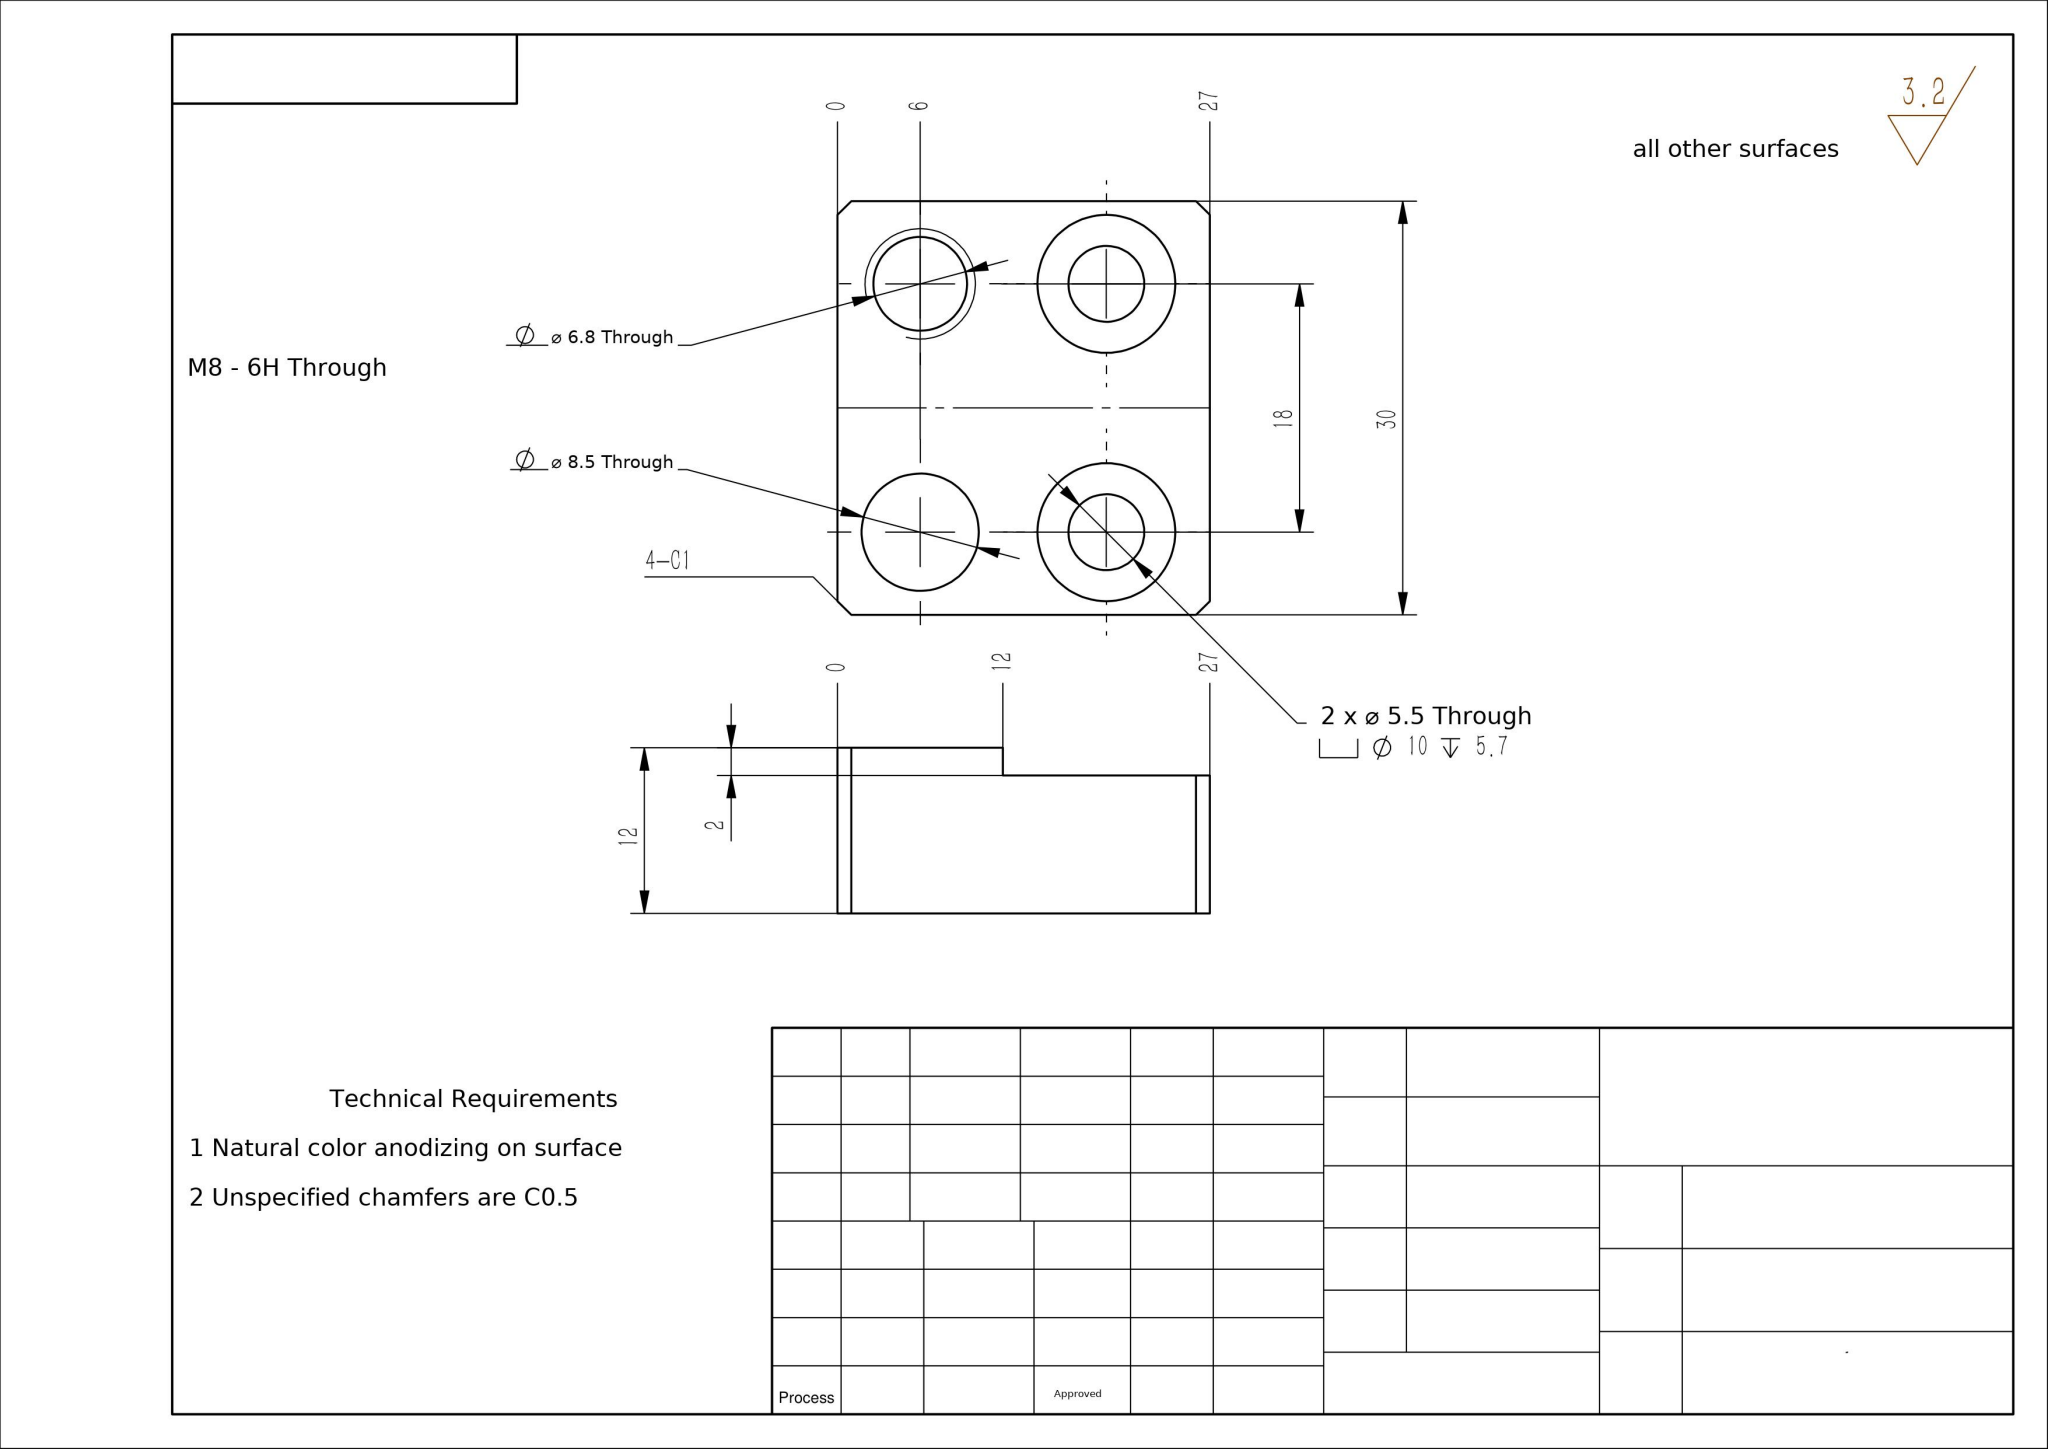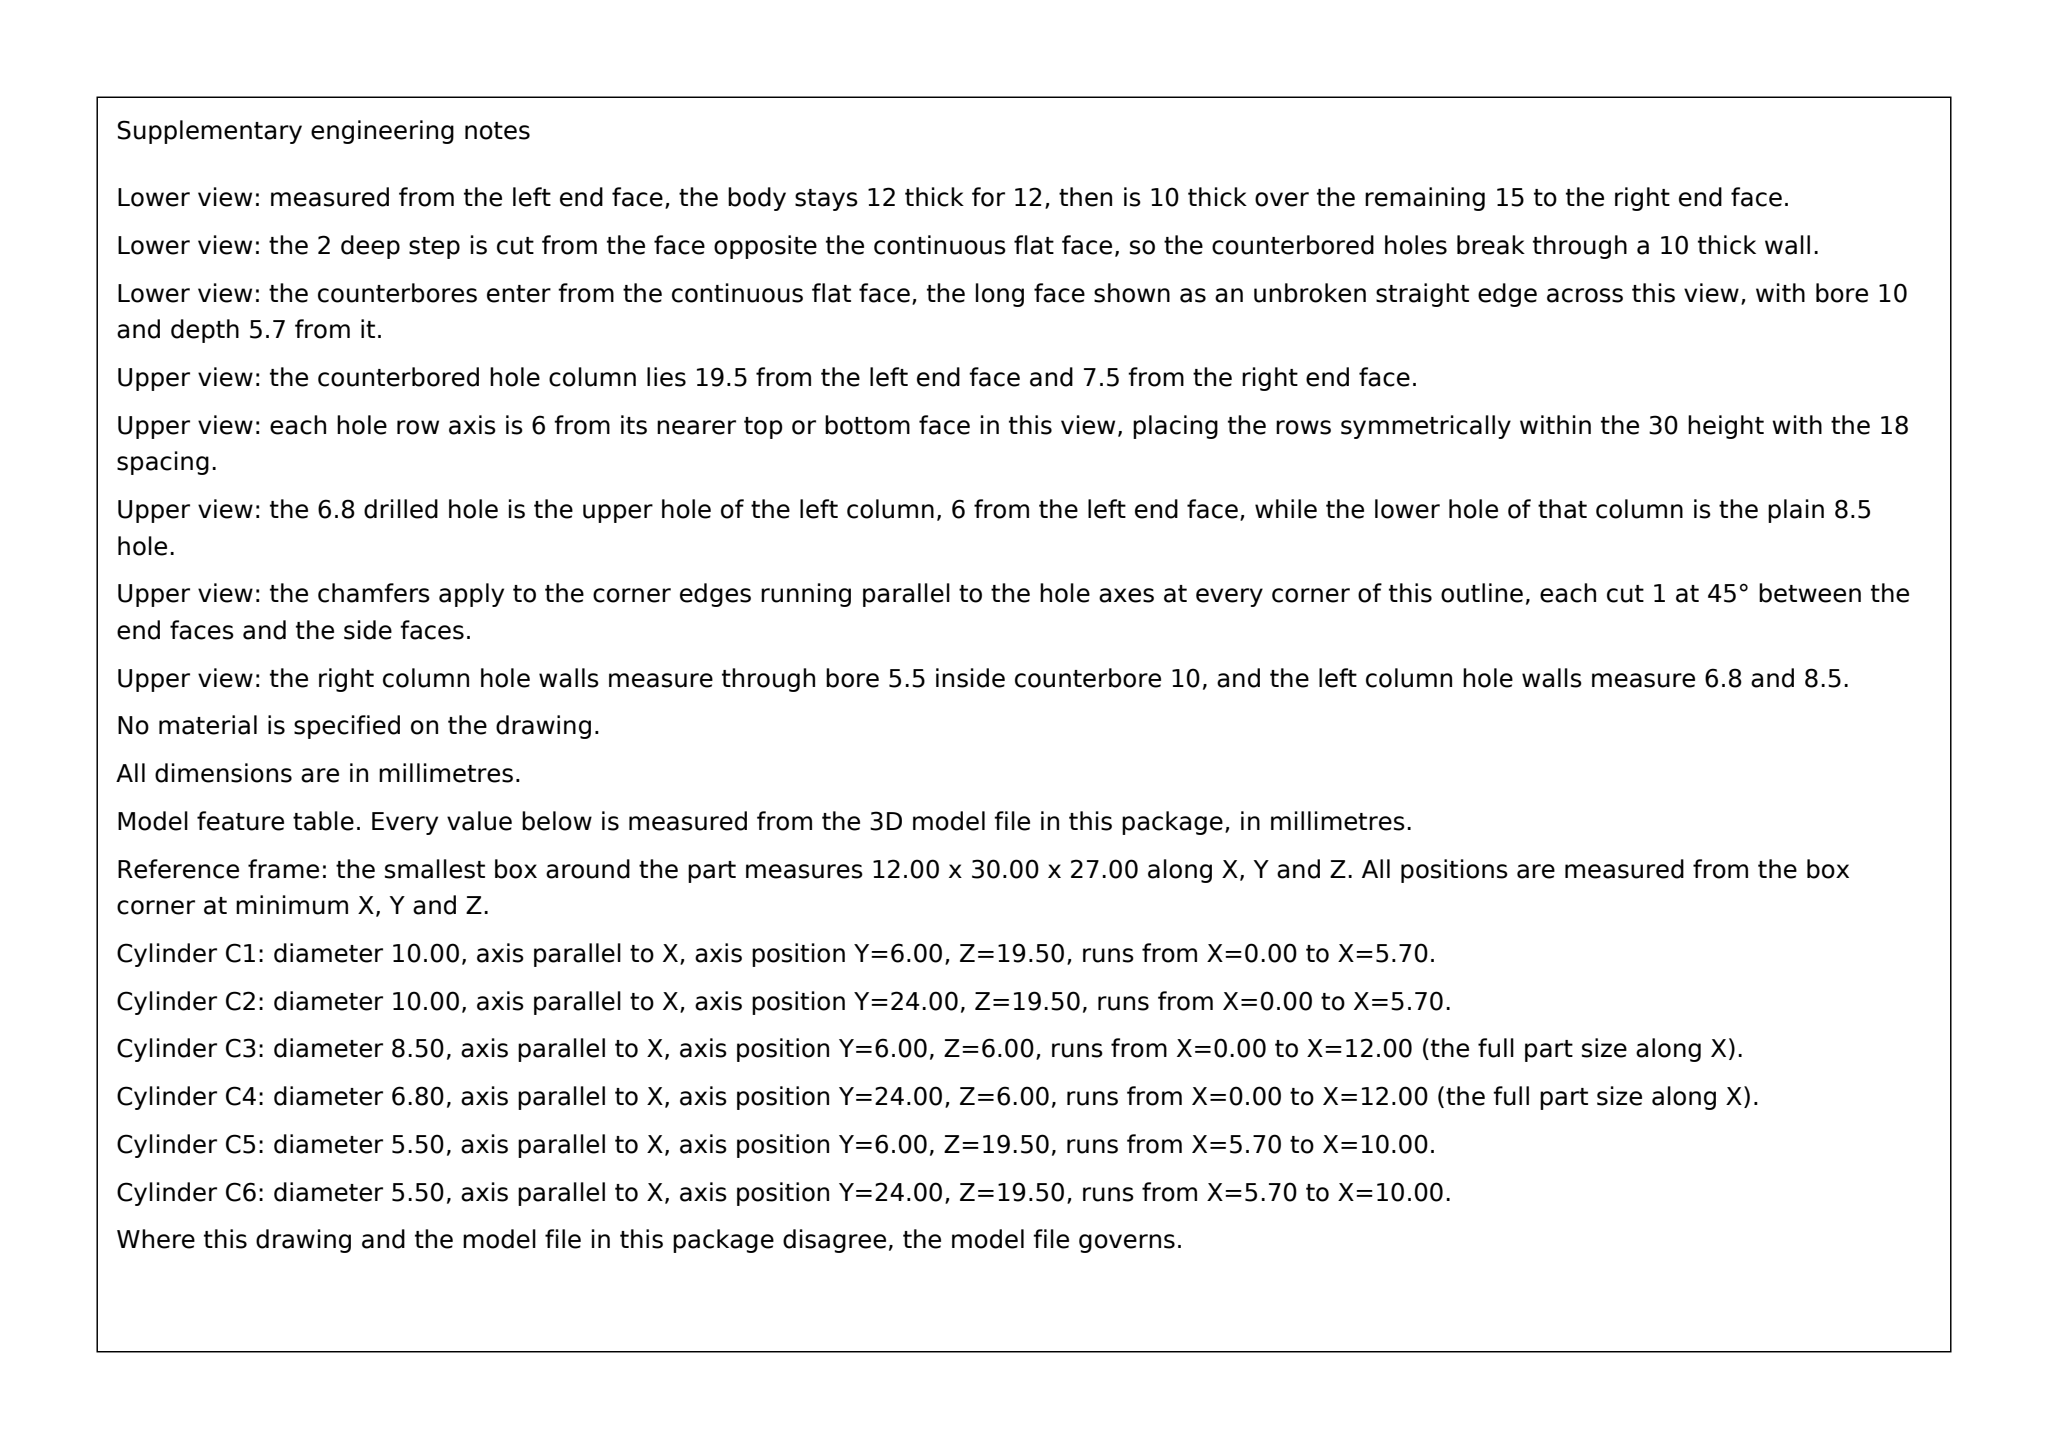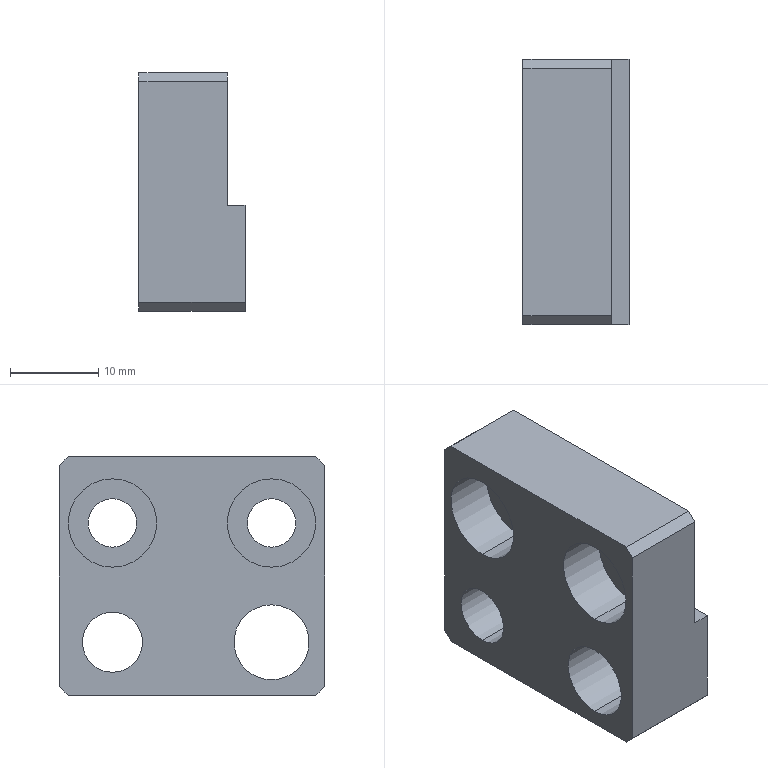Part | SolidWorks | mm | 1 solid | 26 faces | box 12 x 30 x 27 mm | volume 6582 mm3 | plane 14 | cylinder 12 | commonest cylinder face diameters 10 x4 5.5 x4 8.5 x2 6.8 x2
Drawing notes:
2 X Ø5.5/Ø10 C'BORE CL AT ORD 19.5 FROM 0 DATUM EDGE | from the solid: Ø10 & Ø5.5 bores, x-axis, axis_pos z=19.5 (y=6.0 & 24.0); bbox z 0-27
build123d program:
from build123d import *

# Parameters (mm, degrees)
BOSS_EXTRUDE1_DEPTH                               = 30
HOLE_SIZE_ACCORDING_TO_HEXAGON_SOCKET_D           = 5.5
HOLE_SIZE_ACCORDING_TO_HEXAGON_SOCKET_CBORE_D     = 10
HOLE_SIZE_ACCORDING_TO_HEXAGON_SOCKET_CBORE_DEPTH = 5.7
M8_TAPPED_HOLE1_D                                 = 6.8
F_8_5_8_5_DIAMETER_HOLE1_D                        = 8.5
CHAMFER1_SIZE                                     = 1


with BuildPart() as part:
    # Sketch1 → Boss-Extrude1 (new body)
    with BuildSketch(Plane(origin=(0, 0, 0), x_dir=(1, 0, 0), z_dir=(0, 1, 0))):
        Polygon((-23.167, 25.917), (-11.167, 25.917), (-11.167, 13.917), (-13.167, 13.917), (-13.167, -1.083), (-23.167, -1.083), align=None)
    extrude(amount=BOSS_EXTRUDE1_DEPTH)

    # Hole Size _ according to_ Hexagon Socket (through all)
    with Locations(Plane.ZY.offset(23.167)):
        with Locations((-6.417, 6), (-6.417, 24)):
            CounterBoreHole(HOLE_SIZE_ACCORDING_TO_HEXAGON_SOCKET_D / 2, HOLE_SIZE_ACCORDING_TO_HEXAGON_SOCKET_CBORE_D / 2, HOLE_SIZE_ACCORDING_TO_HEXAGON_SOCKET_CBORE_DEPTH)

    # M8 Tapped Hole1 (through all)
    with Locations(Plane.ZY.offset(23.167)):
        with Locations((-19.917, 24)):
            Hole(M8_TAPPED_HOLE1_D / 2)

    # 8.5 _8.5_ Diameter Hole1 (through all)
    with Locations(Plane.ZY.offset(23.167)):
        with Locations((-19.917, 6)):
            Hole(F_8_5_8_5_DIAMETER_HOLE1_D / 2)

    # Chamfer1
    chamfer1_edges = [part.edges().sort_by_distance(p)[0] for p in [
        (-17.167, 30, -25.917),
        (-17.167, 0, -25.917),
        (-18.167, 30, 1.083),
        (-18.167, 0, 1.083),
    ]]
    chamfer(chamfer1_edges, length=CHAMFER1_SIZE)


solid = part.part
STEP:
#1=CARTESIAN_POINT('',(-11.167,6.,-24.167));
#2=VERTEX_POINT('',#1);
#3=CARTESIAN_POINT('',(-11.167,6.,-15.667));
#4=VERTEX_POINT('',#3);
#5=CARTESIAN_POINT('',(-11.167,6.,-19.917));
#6=DIRECTION('',(-1.,0.,0.));
#7=DIRECTION('',(0.,0.,1.));
#8=AXIS2_PLACEMENT_3D('',#5,#6,#7);
#9=CIRCLE('',#8,4.25);
#10=EDGE_CURVE('',#2,#4,#9,.T.);
#11=ORIENTED_EDGE('',*,*,#10,.F.);
#12=CARTESIAN_POINT('',(-23.167,6.,-24.167));
#13=VERTEX_POINT('',#12);
#14=CARTESIAN_POINT('',(-23.167,6.,-24.167));
#15=DIRECTION('',(-1.,0.,0.));
#16=VECTOR('',#15,1000.);
#17=LINE('',#14,#16);
#18=EDGE_CURVE('',#2,#13,#17,.T.);
#19=ORIENTED_EDGE('',*,*,#18,.T.);
#20=CARTESIAN_POINT('',(-23.167,6.,-15.667));
#21=VERTEX_POINT('',#20);
#22=CARTESIAN_POINT('',(-23.167,6.,-19.917));
#23=DIRECTION('',(-1.,0.,0.));
#24=DIRECTION('',(0.,0.,1.));
#25=AXIS2_PLACEMENT_3D('',#22,#23,#24);
#26=CIRCLE('',#25,4.25);
#27=EDGE_CURVE('',#13,#21,#26,.T.);
#28=ORIENTED_EDGE('',*,*,#27,.T.);
#29=CARTESIAN_POINT('',(-23.167,6.,-15.667));
#30=DIRECTION('',(-1.,0.,0.));
#31=VECTOR('',#30,1000.);
#32=LINE('',#29,#31);
#33=EDGE_CURVE('',#4,#21,#32,.T.);
#34=ORIENTED_EDGE('',*,*,#33,.F.);
#35=EDGE_LOOP('',(#11,#19,#28,#34));
#36=FACE_OUTER_BOUND('',#35,.T.);
#37=CARTESIAN_POINT('',(-23.167,6.,-19.917));
#38=DIRECTION('',(-1.,0.,0.));
#39=DIRECTION('',(0.,0.,1.));
#40=AXIS2_PLACEMENT_3D('',#37,#38,#39);
#41=CYLINDRICAL_SURFACE('',#40,4.25);
#42=ADVANCED_FACE('',(#36),#41,.F.);
#43=CARTESIAN_POINT('',(-11.167,24.,-23.317));
#44=VERTEX_POINT('',#43);
#45=CARTESIAN_POINT('',(-11.167,24.,-16.517));
#46=VERTEX_POINT('',#45);
#47=CARTESIAN_POINT('',(-11.167,24.,-19.917));
#48=DIRECTION('',(-1.,0.,0.));
#49=DIRECTION('',(0.,0.,1.));
#50=AXIS2_PLACEMENT_3D('',#47,#48,#49);
#51=CIRCLE('',#50,3.4);
#52=EDGE_CURVE('',#44,#46,#51,.T.);
#53=ORIENTED_EDGE('',*,*,#52,.F.);
#54=CARTESIAN_POINT('',(-23.167,24.,-23.317));
#55=VERTEX_POINT('',#54);
#56=CARTESIAN_POINT('',(-23.167,24.,-23.317));
#57=DIRECTION('',(-1.,0.,0.));
#58=VECTOR('',#57,1000.);
#59=LINE('',#56,#58);
#60=EDGE_CURVE('',#44,#55,#59,.T.);
#61=ORIENTED_EDGE('',*,*,#60,.T.);
#62=CARTESIAN_POINT('',(-23.167,24.,-16.517));
#63=VERTEX_POINT('',#62);
#64=CARTESIAN_POINT('',(-23.167,24.,-19.917));
#65=DIRECTION('',(-1.,0.,0.));
#66=DIRECTION('',(0.,0.,1.));
#67=AXIS2_PLACEMENT_3D('',#64,#65,#66);
#68=CIRCLE('',#67,3.4);
#69=EDGE_CURVE('',#55,#63,#68,.T.);
#70=ORIENTED_EDGE('',*,*,#69,.T.);
#71=CARTESIAN_POINT('',(-23.167,24.,-16.517));
#72=DIRECTION('',(-1.,0.,0.));
#73=VECTOR('',#72,1000.);
#74=LINE('',#71,#73);
#75=EDGE_CURVE('',#46,#63,#74,.T.);
#76=ORIENTED_EDGE('',*,*,#75,.F.);
#77=EDGE_LOOP('',(#53,#61,#70,#76));
#78=FACE_OUTER_BOUND('',#77,.T.);
#79=CARTESIAN_POINT('',(-23.167,24.,-19.917));
#80=DIRECTION('',(-1.,0.,0.));
#81=DIRECTION('',(0.,0.,1.));
#82=AXIS2_PLACEMENT_3D('',#79,#80,#81);
#83=CYLINDRICAL_SURFACE('',#82,3.4);
#84=ADVANCED_FACE('',(#78),#83,.F.);
#85=CARTESIAN_POINT('',(-17.467,6.,-11.417));
#86=VERTEX_POINT('',#85);
#87=CARTESIAN_POINT('',(-17.467,6.,-1.417));
#88=VERTEX_POINT('',#87);
#89=CARTESIAN_POINT('',(-17.467,6.,-6.417));
#90=DIRECTION('',(-1.,0.,0.));
#91=DIRECTION('',(0.,0.,1.));
#92=AXIS2_PLACEMENT_3D('',#89,#90,#91);
#93=CIRCLE('',#92,5.);
#94=EDGE_CURVE('',#86,#88,#93,.T.);
#95=ORIENTED_EDGE('',*,*,#94,.F.);
#96=CARTESIAN_POINT('',(-23.167,6.,-11.417));
#97=VERTEX_POINT('',#96);
#98=CARTESIAN_POINT('',(-23.167,6.,-11.417));
#99=DIRECTION('',(-1.,0.,0.));
#100=VECTOR('',#99,1000.);
#101=LINE('',#98,#100);
#102=EDGE_CURVE('',#86,#97,#101,.T.);
#103=ORIENTED_EDGE('',*,*,#102,.T.);
#104=CARTESIAN_POINT('',(-23.167,6.,-1.417));
#105=VERTEX_POINT('',#104);
#106=CARTESIAN_POINT('',(-23.167,6.,-6.417));
#107=DIRECTION('',(-1.,0.,0.));
#108=DIRECTION('',(0.,0.,1.));
#109=AXIS2_PLACEMENT_3D('',#106,#107,#108);
#110=CIRCLE('',#109,5.);
#111=EDGE_CURVE('',#97,#105,#110,.T.);
#112=ORIENTED_EDGE('',*,*,#111,.T.);
#113=CARTESIAN_POINT('',(-23.167,6.,-1.417));
#114=DIRECTION('',(-1.,0.,0.));
#115=VECTOR('',#114,1000.);
#116=LINE('',#113,#115);
#117=EDGE_CURVE('',#88,#105,#116,.T.);
#118=ORIENTED_EDGE('',*,*,#117,.F.);
#119=EDGE_LOOP('',(#95,#103,#112,#118));
#120=FACE_OUTER_BOUND('',#119,.T.);
#121=CARTESIAN_POINT('',(-23.167,6.,-6.417));
#122=DIRECTION('',(-1.,0.,0.));
#123=DIRECTION('',(0.,0.,1.));
#124=AXIS2_PLACEMENT_3D('',#121,#122,#123);
#125=CYLINDRICAL_SURFACE('',#124,5.);
#126=ADVANCED_FACE('',(#120),#125,.F.);
#127=CARTESIAN_POINT('',(-13.167,6.,-9.167));
#128=VERTEX_POINT('',#127);
#129=CARTESIAN_POINT('',(-13.167,6.,-3.667));
#130=VERTEX_POINT('',#129);
#131=CARTESIAN_POINT('',(-13.167,6.,-6.417));
#132=DIRECTION('',(-1.,0.,0.));
#133=DIRECTION('',(0.,0.,1.));
#134=AXIS2_PLACEMENT_3D('',#131,#132,#133);
#135=CIRCLE('',#134,2.75);
#136=EDGE_CURVE('',#128,#130,#135,.T.);
#137=ORIENTED_EDGE('',*,*,#136,.F.);
#138=CARTESIAN_POINT('',(-17.467,6.,-9.167));
#139=VERTEX_POINT('',#138);
#140=CARTESIAN_POINT('',(-23.167,6.,-9.167));
#141=DIRECTION('',(-1.,0.,0.));
#142=VECTOR('',#141,1000.);
#143=LINE('',#140,#142);
#144=EDGE_CURVE('',#128,#139,#143,.T.);
#145=ORIENTED_EDGE('',*,*,#144,.T.);
#146=CARTESIAN_POINT('',(-17.467,6.,-3.667));
#147=VERTEX_POINT('',#146);
#148=CARTESIAN_POINT('',(-17.467,6.,-6.417));
#149=DIRECTION('',(-1.,0.,0.));
#150=DIRECTION('',(0.,0.,1.));
#151=AXIS2_PLACEMENT_3D('',#148,#149,#150);
#152=CIRCLE('',#151,2.75);
#153=EDGE_CURVE('',#139,#147,#152,.T.);
#154=ORIENTED_EDGE('',*,*,#153,.T.);
#155=CARTESIAN_POINT('',(-23.167,6.,-3.667));
#156=DIRECTION('',(-1.,0.,0.));
#157=VECTOR('',#156,1000.);
#158=LINE('',#155,#157);
#159=EDGE_CURVE('',#130,#147,#158,.T.);
#160=ORIENTED_EDGE('',*,*,#159,.F.);
#161=EDGE_LOOP('',(#137,#145,#154,#160));
#162=FACE_OUTER_BOUND('',#161,.T.);
#163=CARTESIAN_POINT('',(-23.167,6.,-6.417));
#164=DIRECTION('',(-1.,0.,0.));
#165=DIRECTION('',(0.,0.,1.));
#166=AXIS2_PLACEMENT_3D('',#163,#164,#165);
#167=CYLINDRICAL_SURFACE('',#166,2.75);
#168=ADVANCED_FACE('',(#162),#167,.F.);
#169=CARTESIAN_POINT('',(-17.467,24.,-11.417));
#170=VERTEX_POINT('',#169);
#171=CARTESIAN_POINT('',(-17.467,24.,-1.417));
#172=VERTEX_POINT('',#171);
#173=CARTESIAN_POINT('',(-17.467,24.,-6.417));
#174=DIRECTION('',(-1.,0.,0.));
#175=DIRECTION('',(0.,0.,1.));
#176=AXIS2_PLACEMENT_3D('',#173,#174,#175);
#177=CIRCLE('',#176,5.);
#178=EDGE_CURVE('',#170,#172,#177,.T.);
#179=ORIENTED_EDGE('',*,*,#178,.F.);
#180=CARTESIAN_POINT('',(-23.167,24.,-11.417));
#181=VERTEX_POINT('',#180);
#182=CARTESIAN_POINT('',(-23.167,24.,-11.417));
#183=DIRECTION('',(-1.,0.,0.));
#184=VECTOR('',#183,1000.);
#185=LINE('',#182,#184);
#186=EDGE_CURVE('',#170,#181,#185,.T.);
#187=ORIENTED_EDGE('',*,*,#186,.T.);
#188=CARTESIAN_POINT('',(-23.167,24.,-1.417));
#189=VERTEX_POINT('',#188);
#190=CARTESIAN_POINT('',(-23.167,24.,-6.417));
#191=DIRECTION('',(-1.,0.,0.));
#192=DIRECTION('',(0.,0.,1.));
#193=AXIS2_PLACEMENT_3D('',#190,#191,#192);
#194=CIRCLE('',#193,5.);
#195=EDGE_CURVE('',#181,#189,#194,.T.);
#196=ORIENTED_EDGE('',*,*,#195,.T.);
#197=CARTESIAN_POINT('',(-23.167,24.,-1.417));
#198=DIRECTION('',(-1.,0.,0.));
#199=VECTOR('',#198,1000.);
#200=LINE('',#197,#199);
#201=EDGE_CURVE('',#172,#189,#200,.T.);
#202=ORIENTED_EDGE('',*,*,#201,.F.);
#203=EDGE_LOOP('',(#179,#187,#196,#202));
#204=FACE_OUTER_BOUND('',#203,.T.);
#205=CARTESIAN_POINT('',(-23.167,24.,-6.417));
#206=DIRECTION('',(-1.,0.,0.));
#207=DIRECTION('',(0.,0.,1.));
#208=AXIS2_PLACEMENT_3D('',#205,#206,#207);
#209=CYLINDRICAL_SURFACE('',#208,5.);
#210=ADVANCED_FACE('',(#204),#209,.F.);
#211=CARTESIAN_POINT('',(-13.167,24.,-9.167));
#212=VERTEX_POINT('',#211);
#213=CARTESIAN_POINT('',(-13.167,24.,-3.667));
#214=VERTEX_POINT('',#213);
#215=CARTESIAN_POINT('',(-13.167,24.,-6.417));
#216=DIRECTION('',(-1.,0.,0.));
#217=DIRECTION('',(0.,0.,1.));
#218=AXIS2_PLACEMENT_3D('',#215,#216,#217);
#219=CIRCLE('',#218,2.75);
#220=EDGE_CURVE('',#212,#214,#219,.T.);
#221=ORIENTED_EDGE('',*,*,#220,.F.);
#222=CARTESIAN_POINT('',(-17.467,24.,-9.167));
#223=VERTEX_POINT('',#222);
#224=CARTESIAN_POINT('',(-23.167,24.,-9.167));
#225=DIRECTION('',(-1.,0.,0.));
#226=VECTOR('',#225,1000.);
#227=LINE('',#224,#226);
#228=EDGE_CURVE('',#212,#223,#227,.T.);
#229=ORIENTED_EDGE('',*,*,#228,.T.);
#230=CARTESIAN_POINT('',(-17.467,24.,-3.667));
#231=VERTEX_POINT('',#230);
#232=CARTESIAN_POINT('',(-17.467,24.,-6.417));
#233=DIRECTION('',(-1.,0.,0.));
#234=DIRECTION('',(0.,0.,1.));
#235=AXIS2_PLACEMENT_3D('',#232,#233,#234);
#236=CIRCLE('',#235,2.75);
#237=EDGE_CURVE('',#223,#231,#236,.T.);
#238=ORIENTED_EDGE('',*,*,#237,.T.);
#239=CARTESIAN_POINT('',(-23.167,24.,-3.667));
#240=DIRECTION('',(-1.,0.,0.));
#241=VECTOR('',#240,1000.);
#242=LINE('',#239,#241);
#243=EDGE_CURVE('',#214,#231,#242,.T.);
#244=ORIENTED_EDGE('',*,*,#243,.F.);
#245=EDGE_LOOP('',(#221,#229,#238,#244));
#246=FACE_OUTER_BOUND('',#245,.T.);
#247=CARTESIAN_POINT('',(-23.167,24.,-6.417));
#248=DIRECTION('',(-1.,0.,0.));
#249=DIRECTION('',(0.,0.,1.));
#250=AXIS2_PLACEMENT_3D('',#247,#248,#249);
#251=CYLINDRICAL_SURFACE('',#250,2.75);
#252=ADVANCED_FACE('',(#246),#251,.F.);
#253=CARTESIAN_POINT('',(-23.167,6.,-19.917));
#254=DIRECTION('',(-1.,0.,0.));
#255=DIRECTION('',(0.,0.,1.));
#256=AXIS2_PLACEMENT_3D('',#253,#254,#255);
#257=CIRCLE('',#256,4.25);
#258=EDGE_CURVE('',#21,#13,#257,.T.);
#259=ORIENTED_EDGE('',*,*,#258,.F.);
#260=ORIENTED_EDGE('',*,*,#27,.F.);
#261=EDGE_LOOP('',(#259,#260));
#262=FACE_BOUND('',#261,.T.);
#263=CARTESIAN_POINT('',(-23.167,24.,-19.917));
#264=DIRECTION('',(-1.,0.,0.));
#265=DIRECTION('',(0.,0.,1.));
#266=AXIS2_PLACEMENT_3D('',#263,#264,#265);
#267=CIRCLE('',#266,3.4);
#268=EDGE_CURVE('',#63,#55,#267,.T.);
#269=ORIENTED_EDGE('',*,*,#268,.F.);
#270=ORIENTED_EDGE('',*,*,#69,.F.);
#271=EDGE_LOOP('',(#269,#270));
#272=FACE_BOUND('',#271,.T.);
#273=CARTESIAN_POINT('',(-23.167,6.,-6.417));
#274=DIRECTION('',(-1.,0.,0.));
#275=DIRECTION('',(0.,0.,1.));
#276=AXIS2_PLACEMENT_3D('',#273,#274,#275);
#277=CIRCLE('',#276,5.);
#278=EDGE_CURVE('',#105,#97,#277,.T.);
#279=ORIENTED_EDGE('',*,*,#278,.F.);
#280=ORIENTED_EDGE('',*,*,#111,.F.);
#281=EDGE_LOOP('',(#279,#280));
#282=FACE_BOUND('',#281,.T.);
#283=CARTESIAN_POINT('',(-23.167,24.,-6.417));
#284=DIRECTION('',(-1.,0.,0.));
#285=DIRECTION('',(0.,0.,1.));
#286=AXIS2_PLACEMENT_3D('',#283,#284,#285);
#287=CIRCLE('',#286,5.);
#288=EDGE_CURVE('',#189,#181,#287,.T.);
#289=ORIENTED_EDGE('',*,*,#288,.F.);
#290=ORIENTED_EDGE('',*,*,#195,.F.);
#291=EDGE_LOOP('',(#289,#290));
#292=FACE_BOUND('',#291,.T.);
#293=CARTESIAN_POINT('',(-23.167,0.,-24.917));
#294=VERTEX_POINT('',#293);
#295=CARTESIAN_POINT('',(-23.167,0.,0.08333));
#296=VERTEX_POINT('',#295);
#297=CARTESIAN_POINT('',(-23.167,0.,1.083));
#298=DIRECTION('',(0.,0.,1.));
#299=VECTOR('',#298,1000.);
#300=LINE('',#297,#299);
#301=EDGE_CURVE('',#294,#296,#300,.T.);
#302=ORIENTED_EDGE('',*,*,#301,.T.);
#303=CARTESIAN_POINT('',(-23.167,1.,1.083));
#304=VERTEX_POINT('',#303);
#305=CARTESIAN_POINT('',(-23.167,1.,1.083));
#306=DIRECTION('',(0.,0.7071,0.7071));
#307=VECTOR('',#306,1000.);
#308=LINE('',#305,#307);
#309=EDGE_CURVE('',#296,#304,#308,.T.);
#310=ORIENTED_EDGE('',*,*,#309,.T.);
#311=CARTESIAN_POINT('',(-23.167,29.,1.083));
#312=VERTEX_POINT('',#311);
#313=CARTESIAN_POINT('',(-23.167,30.,1.083));
#314=DIRECTION('',(0.,-1.,0.));
#315=VECTOR('',#314,1000.);
#316=LINE('',#313,#315);
#317=EDGE_CURVE('',#312,#304,#316,.T.);
#318=ORIENTED_EDGE('',*,*,#317,.F.);
#319=CARTESIAN_POINT('',(-23.167,30.,0.08333));
#320=VERTEX_POINT('',#319);
#321=CARTESIAN_POINT('',(-23.167,30.,0.08333));
#322=DIRECTION('',(0.,0.7071,-0.7071));
#323=VECTOR('',#322,1000.);
#324=LINE('',#321,#323);
#325=EDGE_CURVE('',#312,#320,#324,.T.);
#326=ORIENTED_EDGE('',*,*,#325,.T.);
#327=CARTESIAN_POINT('',(-23.167,30.,-24.917));
#328=VERTEX_POINT('',#327);
#329=CARTESIAN_POINT('',(-23.167,30.,1.083));
#330=DIRECTION('',(0.,0.,1.));
#331=VECTOR('',#330,1000.);
#332=LINE('',#329,#331);
#333=EDGE_CURVE('',#328,#320,#332,.T.);
#334=ORIENTED_EDGE('',*,*,#333,.F.);
#335=CARTESIAN_POINT('',(-23.167,29.,-25.917));
#336=VERTEX_POINT('',#335);
#337=CARTESIAN_POINT('',(-23.167,30.,-24.917));
#338=DIRECTION('',(0.,-0.7071,-0.7071));
#339=VECTOR('',#338,1000.);
#340=LINE('',#337,#339);
#341=EDGE_CURVE('',#328,#336,#340,.T.);
#342=ORIENTED_EDGE('',*,*,#341,.T.);
#343=CARTESIAN_POINT('',(-23.167,1.,-25.917));
#344=VERTEX_POINT('',#343);
#345=CARTESIAN_POINT('',(-23.167,30.,-25.917));
#346=DIRECTION('',(0.,-1.,0.));
#347=VECTOR('',#346,1000.);
#348=LINE('',#345,#347);
#349=EDGE_CURVE('',#336,#344,#348,.T.);
#350=ORIENTED_EDGE('',*,*,#349,.T.);
#351=CARTESIAN_POINT('',(-23.167,1.,-25.917));
#352=DIRECTION('',(0.,-0.7071,0.7071));
#353=VECTOR('',#352,1000.);
#354=LINE('',#351,#353);
#355=EDGE_CURVE('',#344,#294,#354,.T.);
#356=ORIENTED_EDGE('',*,*,#355,.T.);
#357=EDGE_LOOP('',(#302,#310,#318,#326,#334,#342,#350,#356));
#358=FACE_OUTER_BOUND('',#357,.T.);
#359=CARTESIAN_POINT('',(-23.167,30.,1.083));
#360=DIRECTION('',(1.,0.,0.));
#361=DIRECTION('',(0.,0.,-1.));
#362=AXIS2_PLACEMENT_3D('',#359,#360,#361);
#363=PLANE('',#362);
#364=ADVANCED_FACE('',(#262,#272,#282,#292,#358),#363,.F.);
#365=ORIENTED_EDGE('',*,*,#317,.T.);
#366=CARTESIAN_POINT('',(-13.167,1.,1.083));
#367=VERTEX_POINT('',#366);
#368=CARTESIAN_POINT('',(-13.167,1.,1.083));
#369=DIRECTION('',(1.,0.,-0.));
#370=VECTOR('',#369,1000.);
#371=LINE('',#368,#370);
#372=EDGE_CURVE('',#304,#367,#371,.T.);
#373=ORIENTED_EDGE('',*,*,#372,.T.);
#374=CARTESIAN_POINT('',(-13.167,29.,1.083));
#375=VERTEX_POINT('',#374);
#376=CARTESIAN_POINT('',(-13.167,30.,1.083));
#377=DIRECTION('',(0.,-1.,0.));
#378=VECTOR('',#377,1000.);
#379=LINE('',#376,#378);
#380=EDGE_CURVE('',#375,#367,#379,.T.);
#381=ORIENTED_EDGE('',*,*,#380,.F.);
#382=CARTESIAN_POINT('',(-13.167,29.,1.083));
#383=DIRECTION('',(-1.,0.,0.));
#384=VECTOR('',#383,1000.);
#385=LINE('',#382,#384);
#386=EDGE_CURVE('',#375,#312,#385,.T.);
#387=ORIENTED_EDGE('',*,*,#386,.T.);
#388=EDGE_LOOP('',(#365,#373,#381,#387));
#389=FACE_OUTER_BOUND('',#388,.T.);
#390=CARTESIAN_POINT('',(-13.167,30.,1.083));
#391=DIRECTION('',(-0.,0.,-1.));
#392=DIRECTION('',(-1.,0.,0.));
#393=AXIS2_PLACEMENT_3D('',#390,#391,#392);
#394=PLANE('',#393);
#395=ADVANCED_FACE('',(#389),#394,.F.);
#396=CARTESIAN_POINT('',(-13.167,6.,-6.417));
#397=DIRECTION('',(-1.,0.,0.));
#398=DIRECTION('',(0.,0.,1.));
#399=AXIS2_PLACEMENT_3D('',#396,#397,#398);
#400=CIRCLE('',#399,2.75);
#401=EDGE_CURVE('',#130,#128,#400,.T.);
#402=ORIENTED_EDGE('',*,*,#401,.T.);
#403=ORIENTED_EDGE('',*,*,#136,.T.);
#404=EDGE_LOOP('',(#402,#403));
#405=FACE_BOUND('',#404,.T.);
#406=CARTESIAN_POINT('',(-13.167,24.,-6.417));
#407=DIRECTION('',(-1.,0.,0.));
#408=DIRECTION('',(0.,0.,1.));
#409=AXIS2_PLACEMENT_3D('',#406,#407,#408);
#410=CIRCLE('',#409,2.75);
#411=EDGE_CURVE('',#214,#212,#410,.T.);
#412=ORIENTED_EDGE('',*,*,#411,.T.);
#413=ORIENTED_EDGE('',*,*,#220,.T.);
#414=EDGE_LOOP('',(#412,#413));
#415=FACE_BOUND('',#414,.T.);
#416=ORIENTED_EDGE('',*,*,#380,.T.);
#417=CARTESIAN_POINT('',(-13.167,0.,0.08333));
#418=VERTEX_POINT('',#417);
#419=CARTESIAN_POINT('',(-13.167,1.,1.083));
#420=DIRECTION('',(-0.,-0.7071,-0.7071));
#421=VECTOR('',#420,1000.);
#422=LINE('',#419,#421);
#423=EDGE_CURVE('',#367,#418,#422,.T.);
#424=ORIENTED_EDGE('',*,*,#423,.T.);
#425=CARTESIAN_POINT('',(-13.167,0.,-13.917));
#426=VERTEX_POINT('',#425);
#427=CARTESIAN_POINT('',(-13.167,0.,-13.917));
#428=DIRECTION('',(-0.,0.,-1.));
#429=VECTOR('',#428,1000.);
#430=LINE('',#427,#429);
#431=EDGE_CURVE('',#418,#426,#430,.T.);
#432=ORIENTED_EDGE('',*,*,#431,.T.);
#433=CARTESIAN_POINT('',(-13.167,30.,-13.917));
#434=VERTEX_POINT('',#433);
#435=CARTESIAN_POINT('',(-13.167,30.,-13.917));
#436=DIRECTION('',(0.,-1.,0.));
#437=VECTOR('',#436,1000.);
#438=LINE('',#435,#437);
#439=EDGE_CURVE('',#434,#426,#438,.T.);
#440=ORIENTED_EDGE('',*,*,#439,.F.);
#441=CARTESIAN_POINT('',(-13.167,30.,0.08333));
#442=VERTEX_POINT('',#441);
#443=CARTESIAN_POINT('',(-13.167,30.,-13.917));
#444=DIRECTION('',(-0.,0.,-1.));
#445=VECTOR('',#444,1000.);
#446=LINE('',#443,#445);
#447=EDGE_CURVE('',#442,#434,#446,.T.);
#448=ORIENTED_EDGE('',*,*,#447,.F.);
#449=CARTESIAN_POINT('',(-13.167,30.,0.08333));
#450=DIRECTION('',(0.,-0.7071,0.7071));
#451=VECTOR('',#450,1000.);
#452=LINE('',#449,#451);
#453=EDGE_CURVE('',#442,#375,#452,.T.);
#454=ORIENTED_EDGE('',*,*,#453,.T.);
#455=EDGE_LOOP('',(#416,#424,#432,#440,#448,#454));
#456=FACE_OUTER_BOUND('',#455,.T.);
#457=CARTESIAN_POINT('',(-13.167,30.,-13.917));
#458=DIRECTION('',(-1.,0.,0.));
#459=DIRECTION('',(0.,0.,1.));
#460=AXIS2_PLACEMENT_3D('',#457,#458,#459);
#461=PLANE('',#460);
#462=ADVANCED_FACE('',(#405,#415,#456),#461,.F.);
#463=CARTESIAN_POINT('',(-11.167,0.,-13.917));
#464=VERTEX_POINT('',#463);
#465=CARTESIAN_POINT('',(-11.167,0.,-13.917));
#466=DIRECTION('',(1.,0.,0.));
#467=VECTOR('',#466,1000.);
#468=LINE('',#465,#467);
#469=EDGE_CURVE('',#426,#464,#468,.T.);
#470=ORIENTED_EDGE('',*,*,#469,.T.);
#471=CARTESIAN_POINT('',(-11.167,30.,-13.917));
#472=VERTEX_POINT('',#471);
#473=CARTESIAN_POINT('',(-11.167,30.,-13.917));
#474=DIRECTION('',(0.,-1.,0.));
#475=VECTOR('',#474,1000.);
#476=LINE('',#473,#475);
#477=EDGE_CURVE('',#472,#464,#476,.T.);
#478=ORIENTED_EDGE('',*,*,#477,.F.);
#479=CARTESIAN_POINT('',(-11.167,30.,-13.917));
#480=DIRECTION('',(1.,0.,0.));
#481=VECTOR('',#480,1000.);
#482=LINE('',#479,#481);
#483=EDGE_CURVE('',#434,#472,#482,.T.);
#484=ORIENTED_EDGE('',*,*,#483,.F.);
#485=ORIENTED_EDGE('',*,*,#439,.T.);
#486=EDGE_LOOP('',(#470,#478,#484,#485));
#487=FACE_OUTER_BOUND('',#486,.T.);
#488=CARTESIAN_POINT('',(-11.167,30.,-13.917));
#489=DIRECTION('',(0.,0.,-1.));
#490=DIRECTION('',(-1.,0.,0.));
#491=AXIS2_PLACEMENT_3D('',#488,#489,#490);
#492=PLANE('',#491);
#493=ADVANCED_FACE('',(#487),#492,.F.);
#494=CARTESIAN_POINT('',(-11.167,6.,-19.917));
#495=DIRECTION('',(-1.,0.,0.));
#496=DIRECTION('',(0.,0.,1.));
#497=AXIS2_PLACEMENT_3D('',#494,#495,#496);
#498=CIRCLE('',#497,4.25);
#499=EDGE_CURVE('',#4,#2,#498,.T.);
#500=ORIENTED_EDGE('',*,*,#499,.T.);
#501=ORIENTED_EDGE('',*,*,#10,.T.);
#502=EDGE_LOOP('',(#500,#501));
#503=FACE_BOUND('',#502,.T.);
#504=CARTESIAN_POINT('',(-11.167,24.,-19.917));
#505=DIRECTION('',(-1.,0.,0.));
#506=DIRECTION('',(0.,0.,1.));
#507=AXIS2_PLACEMENT_3D('',#504,#505,#506);
#508=CIRCLE('',#507,3.4);
#509=EDGE_CURVE('',#46,#44,#508,.T.);
#510=ORIENTED_EDGE('',*,*,#509,.T.);
#511=ORIENTED_EDGE('',*,*,#52,.T.);
#512=EDGE_LOOP('',(#510,#511));
#513=FACE_BOUND('',#512,.T.);
#514=CARTESIAN_POINT('',(-11.167,29.,-25.917));
#515=VERTEX_POINT('',#514);
#516=CARTESIAN_POINT('',(-11.167,1.,-25.917));
#517=VERTEX_POINT('',#516);
#518=CARTESIAN_POINT('',(-11.167,30.,-25.917));
#519=DIRECTION('',(0.,-1.,0.));
#520=VECTOR('',#519,1000.);
#521=LINE('',#518,#520);
#522=EDGE_CURVE('',#515,#517,#521,.T.);
#523=ORIENTED_EDGE('',*,*,#522,.F.);
#524=CARTESIAN_POINT('',(-11.167,30.,-24.917));
#525=VERTEX_POINT('',#524);
#526=CARTESIAN_POINT('',(-11.167,30.,-24.917));
#527=DIRECTION('',(0.,0.7071,0.7071));
#528=VECTOR('',#527,1000.);
#529=LINE('',#526,#528);
#530=EDGE_CURVE('',#515,#525,#529,.T.);
#531=ORIENTED_EDGE('',*,*,#530,.T.);
#532=CARTESIAN_POINT('',(-11.167,30.,-25.917));
#533=DIRECTION('',(-0.,0.,-1.));
#534=VECTOR('',#533,1000.);
#535=LINE('',#532,#534);
#536=EDGE_CURVE('',#472,#525,#535,.T.);
#537=ORIENTED_EDGE('',*,*,#536,.F.);
#538=ORIENTED_EDGE('',*,*,#477,.T.);
#539=CARTESIAN_POINT('',(-11.167,0.,-24.917));
#540=VERTEX_POINT('',#539);
#541=CARTESIAN_POINT('',(-11.167,0.,-25.917));
#542=DIRECTION('',(-0.,0.,-1.));
#543=VECTOR('',#542,1000.);
#544=LINE('',#541,#543);
#545=EDGE_CURVE('',#464,#540,#544,.T.);
#546=ORIENTED_EDGE('',*,*,#545,.T.);
#547=CARTESIAN_POINT('',(-11.167,1.,-25.917));
#548=DIRECTION('',(-0.,0.7071,-0.7071));
#549=VECTOR('',#548,1000.);
#550=LINE('',#547,#549);
#551=EDGE_CURVE('',#540,#517,#550,.T.);
#552=ORIENTED_EDGE('',*,*,#551,.T.);
#553=EDGE_LOOP('',(#523,#531,#537,#538,#546,#552));
#554=FACE_OUTER_BOUND('',#553,.T.);
#555=CARTESIAN_POINT('',(-11.167,30.,-25.917));
#556=DIRECTION('',(-1.,0.,0.));
#557=DIRECTION('',(0.,0.,1.));
#558=AXIS2_PLACEMENT_3D('',#555,#556,#557);
#559=PLANE('',#558);
#560=ADVANCED_FACE('',(#503,#513,#554),#559,.F.);
#561=ORIENTED_EDGE('',*,*,#349,.F.);
#562=CARTESIAN_POINT('',(-23.167,29.,-25.917));
#563=DIRECTION('',(1.,0.,0.));
#564=VECTOR('',#563,1000.);
#565=LINE('',#562,#564);
#566=EDGE_CURVE('',#336,#515,#565,.T.);
#567=ORIENTED_EDGE('',*,*,#566,.T.);
#568=ORIENTED_EDGE('',*,*,#522,.T.);
#569=CARTESIAN_POINT('',(-23.167,1.,-25.917));
#570=DIRECTION('',(-1.,0.,0.));
#571=VECTOR('',#570,1000.);
#572=LINE('',#569,#571);
#573=EDGE_CURVE('',#517,#344,#572,.T.);
#574=ORIENTED_EDGE('',*,*,#573,.T.);
#575=EDGE_LOOP('',(#561,#567,#568,#574));
#576=FACE_OUTER_BOUND('',#575,.T.);
#577=CARTESIAN_POINT('',(-23.167,30.,-25.917));
#578=DIRECTION('',(0.,0.,1.));
#579=DIRECTION('',(1.,0.,0.));
#580=AXIS2_PLACEMENT_3D('',#577,#578,#579);
#581=PLANE('',#580);
#582=ADVANCED_FACE('',(#576),#581,.F.);
#583=ORIENTED_EDGE('',*,*,#333,.T.);
#584=CARTESIAN_POINT('',(0.,30.,0.08333));
#585=DIRECTION('',(1.,0.,-0.));
#586=VECTOR('',#585,1000.);
#587=LINE('',#584,#586);
#588=EDGE_CURVE('',#320,#442,#587,.T.);
#589=ORIENTED_EDGE('',*,*,#588,.T.);
#590=ORIENTED_EDGE('',*,*,#447,.T.);
#591=ORIENTED_EDGE('',*,*,#483,.T.);
#592=ORIENTED_EDGE('',*,*,#536,.T.);
#593=CARTESIAN_POINT('',(0.,30.,-24.917));
#594=DIRECTION('',(-1.,0.,0.));
#595=VECTOR('',#594,1000.);
#596=LINE('',#593,#595);
#597=EDGE_CURVE('',#525,#328,#596,.T.);
#598=ORIENTED_EDGE('',*,*,#597,.T.);
#599=EDGE_LOOP('',(#583,#589,#590,#591,#592,#598));
#600=FACE_OUTER_BOUND('',#599,.T.);
#601=CARTESIAN_POINT('',(0.,30.,0.));
#602=DIRECTION('',(0.,-1.,0.));
#603=DIRECTION('',(0.,0.,-1.));
#604=AXIS2_PLACEMENT_3D('',#601,#602,#603);
#605=PLANE('',#604);
#606=ADVANCED_FACE('',(#600),#605,.F.);
#607=ORIENTED_EDGE('',*,*,#431,.F.);
#608=CARTESIAN_POINT('',(-23.167,0.,0.08333));
#609=DIRECTION('',(-1.,0.,0.));
#610=VECTOR('',#609,1000.);
#611=LINE('',#608,#610);
#612=EDGE_CURVE('',#418,#296,#611,.T.);
#613=ORIENTED_EDGE('',*,*,#612,.T.);
#614=ORIENTED_EDGE('',*,*,#301,.F.);
#615=CARTESIAN_POINT('',(-11.167,0.,-24.917));
#616=DIRECTION('',(1.,0.,0.));
#617=VECTOR('',#616,1000.);
#618=LINE('',#615,#617);
#619=EDGE_CURVE('',#294,#540,#618,.T.);
#620=ORIENTED_EDGE('',*,*,#619,.T.);
#621=ORIENTED_EDGE('',*,*,#545,.F.);
#622=ORIENTED_EDGE('',*,*,#469,.F.);
#623=EDGE_LOOP('',(#607,#613,#614,#620,#621,#622));
#624=FACE_OUTER_BOUND('',#623,.T.);
#625=CARTESIAN_POINT('',(0.,0.,0.));
#626=DIRECTION('',(0.,-1.,0.));
#627=DIRECTION('',(0.,0.,-1.));
#628=AXIS2_PLACEMENT_3D('',#625,#626,#627);
#629=PLANE('',#628);
#630=ADVANCED_FACE('',(#624),#629,.T.);
#631=ORIENTED_EDGE('',*,*,#228,.F.);
#632=ORIENTED_EDGE('',*,*,#411,.F.);
#633=ORIENTED_EDGE('',*,*,#243,.T.);
#634=CARTESIAN_POINT('',(-17.467,24.,-6.417));
#635=DIRECTION('',(-1.,0.,0.));
#636=DIRECTION('',(0.,0.,1.));
#637=AXIS2_PLACEMENT_3D('',#634,#635,#636);
#638=CIRCLE('',#637,2.75);
#639=EDGE_CURVE('',#231,#223,#638,.T.);
#640=ORIENTED_EDGE('',*,*,#639,.T.);
#641=EDGE_LOOP('',(#631,#632,#633,#640));
#642=FACE_OUTER_BOUND('',#641,.T.);
#643=CARTESIAN_POINT('',(-23.167,24.,-6.417));
#644=DIRECTION('',(-1.,0.,0.));
#645=DIRECTION('',(0.,0.,1.));
#646=AXIS2_PLACEMENT_3D('',#643,#644,#645);
#647=CYLINDRICAL_SURFACE('',#646,2.75);
#648=ADVANCED_FACE('',(#642),#647,.F.);
#649=ORIENTED_EDGE('',*,*,#639,.F.);
#650=ORIENTED_EDGE('',*,*,#237,.F.);
#651=EDGE_LOOP('',(#649,#650));
#652=FACE_BOUND('',#651,.T.);
#653=CARTESIAN_POINT('',(-17.467,24.,-6.417));
#654=DIRECTION('',(-1.,0.,0.));
#655=DIRECTION('',(0.,0.,1.));
#656=AXIS2_PLACEMENT_3D('',#653,#654,#655);
#657=CIRCLE('',#656,5.);
#658=EDGE_CURVE('',#172,#170,#657,.T.);
#659=ORIENTED_EDGE('',*,*,#658,.T.);
#660=ORIENTED_EDGE('',*,*,#178,.T.);
#661=EDGE_LOOP('',(#659,#660));
#662=FACE_OUTER_BOUND('',#661,.T.);
#663=CARTESIAN_POINT('',(-17.467,26.75,-6.417));
#664=DIRECTION('',(1.,0.,0.));
#665=DIRECTION('',(0.,0.,-1.));
#666=AXIS2_PLACEMENT_3D('',#663,#664,#665);
#667=PLANE('',#666);
#668=ADVANCED_FACE('',(#652,#662),#667,.F.);
#669=ORIENTED_EDGE('',*,*,#186,.F.);
#670=ORIENTED_EDGE('',*,*,#658,.F.);
#671=ORIENTED_EDGE('',*,*,#201,.T.);
#672=ORIENTED_EDGE('',*,*,#288,.T.);
#673=EDGE_LOOP('',(#669,#670,#671,#672));
#674=FACE_OUTER_BOUND('',#673,.T.);
#675=CARTESIAN_POINT('',(-23.167,24.,-6.417));
#676=DIRECTION('',(-1.,0.,0.));
#677=DIRECTION('',(0.,0.,1.));
#678=AXIS2_PLACEMENT_3D('',#675,#676,#677);
#679=CYLINDRICAL_SURFACE('',#678,5.);
#680=ADVANCED_FACE('',(#674),#679,.F.);
#681=ORIENTED_EDGE('',*,*,#144,.F.);
#682=ORIENTED_EDGE('',*,*,#401,.F.);
#683=ORIENTED_EDGE('',*,*,#159,.T.);
#684=CARTESIAN_POINT('',(-17.467,6.,-6.417));
#685=DIRECTION('',(-1.,0.,0.));
#686=DIRECTION('',(0.,0.,1.));
#687=AXIS2_PLACEMENT_3D('',#684,#685,#686);
#688=CIRCLE('',#687,2.75);
#689=EDGE_CURVE('',#147,#139,#688,.T.);
#690=ORIENTED_EDGE('',*,*,#689,.T.);
#691=EDGE_LOOP('',(#681,#682,#683,#690));
#692=FACE_OUTER_BOUND('',#691,.T.);
#693=CARTESIAN_POINT('',(-23.167,6.,-6.417));
#694=DIRECTION('',(-1.,0.,0.));
#695=DIRECTION('',(0.,0.,1.));
#696=AXIS2_PLACEMENT_3D('',#693,#694,#695);
#697=CYLINDRICAL_SURFACE('',#696,2.75);
#698=ADVANCED_FACE('',(#692),#697,.F.);
#699=ORIENTED_EDGE('',*,*,#689,.F.);
#700=ORIENTED_EDGE('',*,*,#153,.F.);
#701=EDGE_LOOP('',(#699,#700));
#702=FACE_BOUND('',#701,.T.);
#703=CARTESIAN_POINT('',(-17.467,6.,-6.417));
#704=DIRECTION('',(-1.,0.,0.));
#705=DIRECTION('',(0.,0.,1.));
#706=AXIS2_PLACEMENT_3D('',#703,#704,#705);
#707=CIRCLE('',#706,5.);
#708=EDGE_CURVE('',#88,#86,#707,.T.);
#709=ORIENTED_EDGE('',*,*,#708,.T.);
#710=ORIENTED_EDGE('',*,*,#94,.T.);
#711=EDGE_LOOP('',(#709,#710));
#712=FACE_OUTER_BOUND('',#711,.T.);
#713=CARTESIAN_POINT('',(-17.467,8.75,-6.417));
#714=DIRECTION('',(1.,0.,0.));
#715=DIRECTION('',(0.,0.,-1.));
#716=AXIS2_PLACEMENT_3D('',#713,#714,#715);
#717=PLANE('',#716);
#718=ADVANCED_FACE('',(#702,#712),#717,.F.);
#719=ORIENTED_EDGE('',*,*,#102,.F.);
#720=ORIENTED_EDGE('',*,*,#708,.F.);
#721=ORIENTED_EDGE('',*,*,#117,.T.);
#722=ORIENTED_EDGE('',*,*,#278,.T.);
#723=EDGE_LOOP('',(#719,#720,#721,#722));
#724=FACE_OUTER_BOUND('',#723,.T.);
#725=CARTESIAN_POINT('',(-23.167,6.,-6.417));
#726=DIRECTION('',(-1.,0.,0.));
#727=DIRECTION('',(0.,0.,1.));
#728=AXIS2_PLACEMENT_3D('',#725,#726,#727);
#729=CYLINDRICAL_SURFACE('',#728,5.);
#730=ADVANCED_FACE('',(#724),#729,.F.);
#731=ORIENTED_EDGE('',*,*,#60,.F.);
#732=ORIENTED_EDGE('',*,*,#509,.F.);
#733=ORIENTED_EDGE('',*,*,#75,.T.);
#734=ORIENTED_EDGE('',*,*,#268,.T.);
#735=EDGE_LOOP('',(#731,#732,#733,#734));
#736=FACE_OUTER_BOUND('',#735,.T.);
#737=CARTESIAN_POINT('',(-23.167,24.,-19.917));
#738=DIRECTION('',(-1.,0.,0.));
#739=DIRECTION('',(0.,0.,1.));
#740=AXIS2_PLACEMENT_3D('',#737,#738,#739);
#741=CYLINDRICAL_SURFACE('',#740,3.4);
#742=ADVANCED_FACE('',(#736),#741,.F.);
#743=ORIENTED_EDGE('',*,*,#18,.F.);
#744=ORIENTED_EDGE('',*,*,#499,.F.);
#745=ORIENTED_EDGE('',*,*,#33,.T.);
#746=ORIENTED_EDGE('',*,*,#258,.T.);
#747=EDGE_LOOP('',(#743,#744,#745,#746));
#748=FACE_OUTER_BOUND('',#747,.T.);
#749=CARTESIAN_POINT('',(-23.167,6.,-19.917));
#750=DIRECTION('',(-1.,0.,0.));
#751=DIRECTION('',(0.,0.,1.));
#752=AXIS2_PLACEMENT_3D('',#749,#750,#751);
#753=CYLINDRICAL_SURFACE('',#752,4.25);
#754=ADVANCED_FACE('',(#748),#753,.F.);
#755=ORIENTED_EDGE('',*,*,#309,.F.);
#756=ORIENTED_EDGE('',*,*,#612,.F.);
#757=ORIENTED_EDGE('',*,*,#423,.F.);
#758=ORIENTED_EDGE('',*,*,#372,.F.);
#759=EDGE_LOOP('',(#755,#756,#757,#758));
#760=FACE_OUTER_BOUND('',#759,.T.);
#761=CARTESIAN_POINT('',(-13.167,1.,1.083));
#762=DIRECTION('',(0.,-0.7071,0.7071));
#763=DIRECTION('',(-1.,0.,0.));
#764=AXIS2_PLACEMENT_3D('',#761,#762,#763);
#765=PLANE('',#764);
#766=ADVANCED_FACE('',(#760),#765,.T.);
#767=ORIENTED_EDGE('',*,*,#325,.F.);
#768=ORIENTED_EDGE('',*,*,#386,.F.);
#769=ORIENTED_EDGE('',*,*,#453,.F.);
#770=ORIENTED_EDGE('',*,*,#588,.F.);
#771=EDGE_LOOP('',(#767,#768,#769,#770));
#772=FACE_OUTER_BOUND('',#771,.T.);
#773=CARTESIAN_POINT('',(0.,30.,0.08333));
#774=DIRECTION('',(-0.,-0.7071,-0.7071));
#775=DIRECTION('',(1.,0.,-0.));
#776=AXIS2_PLACEMENT_3D('',#773,#774,#775);
#777=PLANE('',#776);
#778=ADVANCED_FACE('',(#772),#777,.F.);
#779=ORIENTED_EDGE('',*,*,#530,.F.);
#780=ORIENTED_EDGE('',*,*,#566,.F.);
#781=ORIENTED_EDGE('',*,*,#341,.F.);
#782=ORIENTED_EDGE('',*,*,#597,.F.);
#783=EDGE_LOOP('',(#779,#780,#781,#782));
#784=FACE_OUTER_BOUND('',#783,.T.);
#785=CARTESIAN_POINT('',(0.,30.,-24.917));
#786=DIRECTION('',(0.,-0.7071,0.7071));
#787=DIRECTION('',(-1.,0.,0.));
#788=AXIS2_PLACEMENT_3D('',#785,#786,#787);
#789=PLANE('',#788);
#790=ADVANCED_FACE('',(#784),#789,.F.);
#791=ORIENTED_EDGE('',*,*,#551,.F.);
#792=ORIENTED_EDGE('',*,*,#619,.F.);
#793=ORIENTED_EDGE('',*,*,#355,.F.);
#794=ORIENTED_EDGE('',*,*,#573,.F.);
#795=EDGE_LOOP('',(#791,#792,#793,#794));
#796=FACE_OUTER_BOUND('',#795,.T.);
#797=CARTESIAN_POINT('',(-23.167,1.,-25.917));
#798=DIRECTION('',(0.,-0.7071,-0.7071));
#799=DIRECTION('',(1.,0.,0.));
#800=AXIS2_PLACEMENT_3D('',#797,#798,#799);
#801=PLANE('',#800);
#802=ADVANCED_FACE('',(#796),#801,.T.);
#803=CLOSED_SHELL('',(#42,#84,#126,#168,#210,#252,#364,#395,#462,#493,#560,#582,#606,#630,#648,#668,#680,#698,#718,#730,#742,#754,#766,#778,#790,#802));
#804=MANIFOLD_SOLID_BREP('',#803);
#805=CARTESIAN_POINT('',(0.,0.,0.));
#806=DIRECTION('',(0.,0.,1.));
#807=DIRECTION('',(1.,0.,0.));
#808=AXIS2_PLACEMENT_3D('',#805,#806,#807);
#809=(LENGTH_UNIT()NAMED_UNIT(*)SI_UNIT(.MILLI.,.METRE.));
#810=UNCERTAINTY_MEASURE_WITH_UNIT(LENGTH_MEASURE(0.00001),#809,'','');
#811=(NAMED_UNIT(*)PLANE_ANGLE_UNIT()SI_UNIT($,.RADIAN.));
#812=(NAMED_UNIT(*)SI_UNIT($,.STERADIAN.)SOLID_ANGLE_UNIT());
#813=(GEOMETRIC_REPRESENTATION_CONTEXT(3)GLOBAL_UNCERTAINTY_ASSIGNED_CONTEXT((#810))GLOBAL_UNIT_ASSIGNED_CONTEXT((#809,#811,#812))REPRESENTATION_CONTEXT('',''));
#814=ADVANCED_BREP_SHAPE_REPRESENTATION('',(#804,#808),#813);